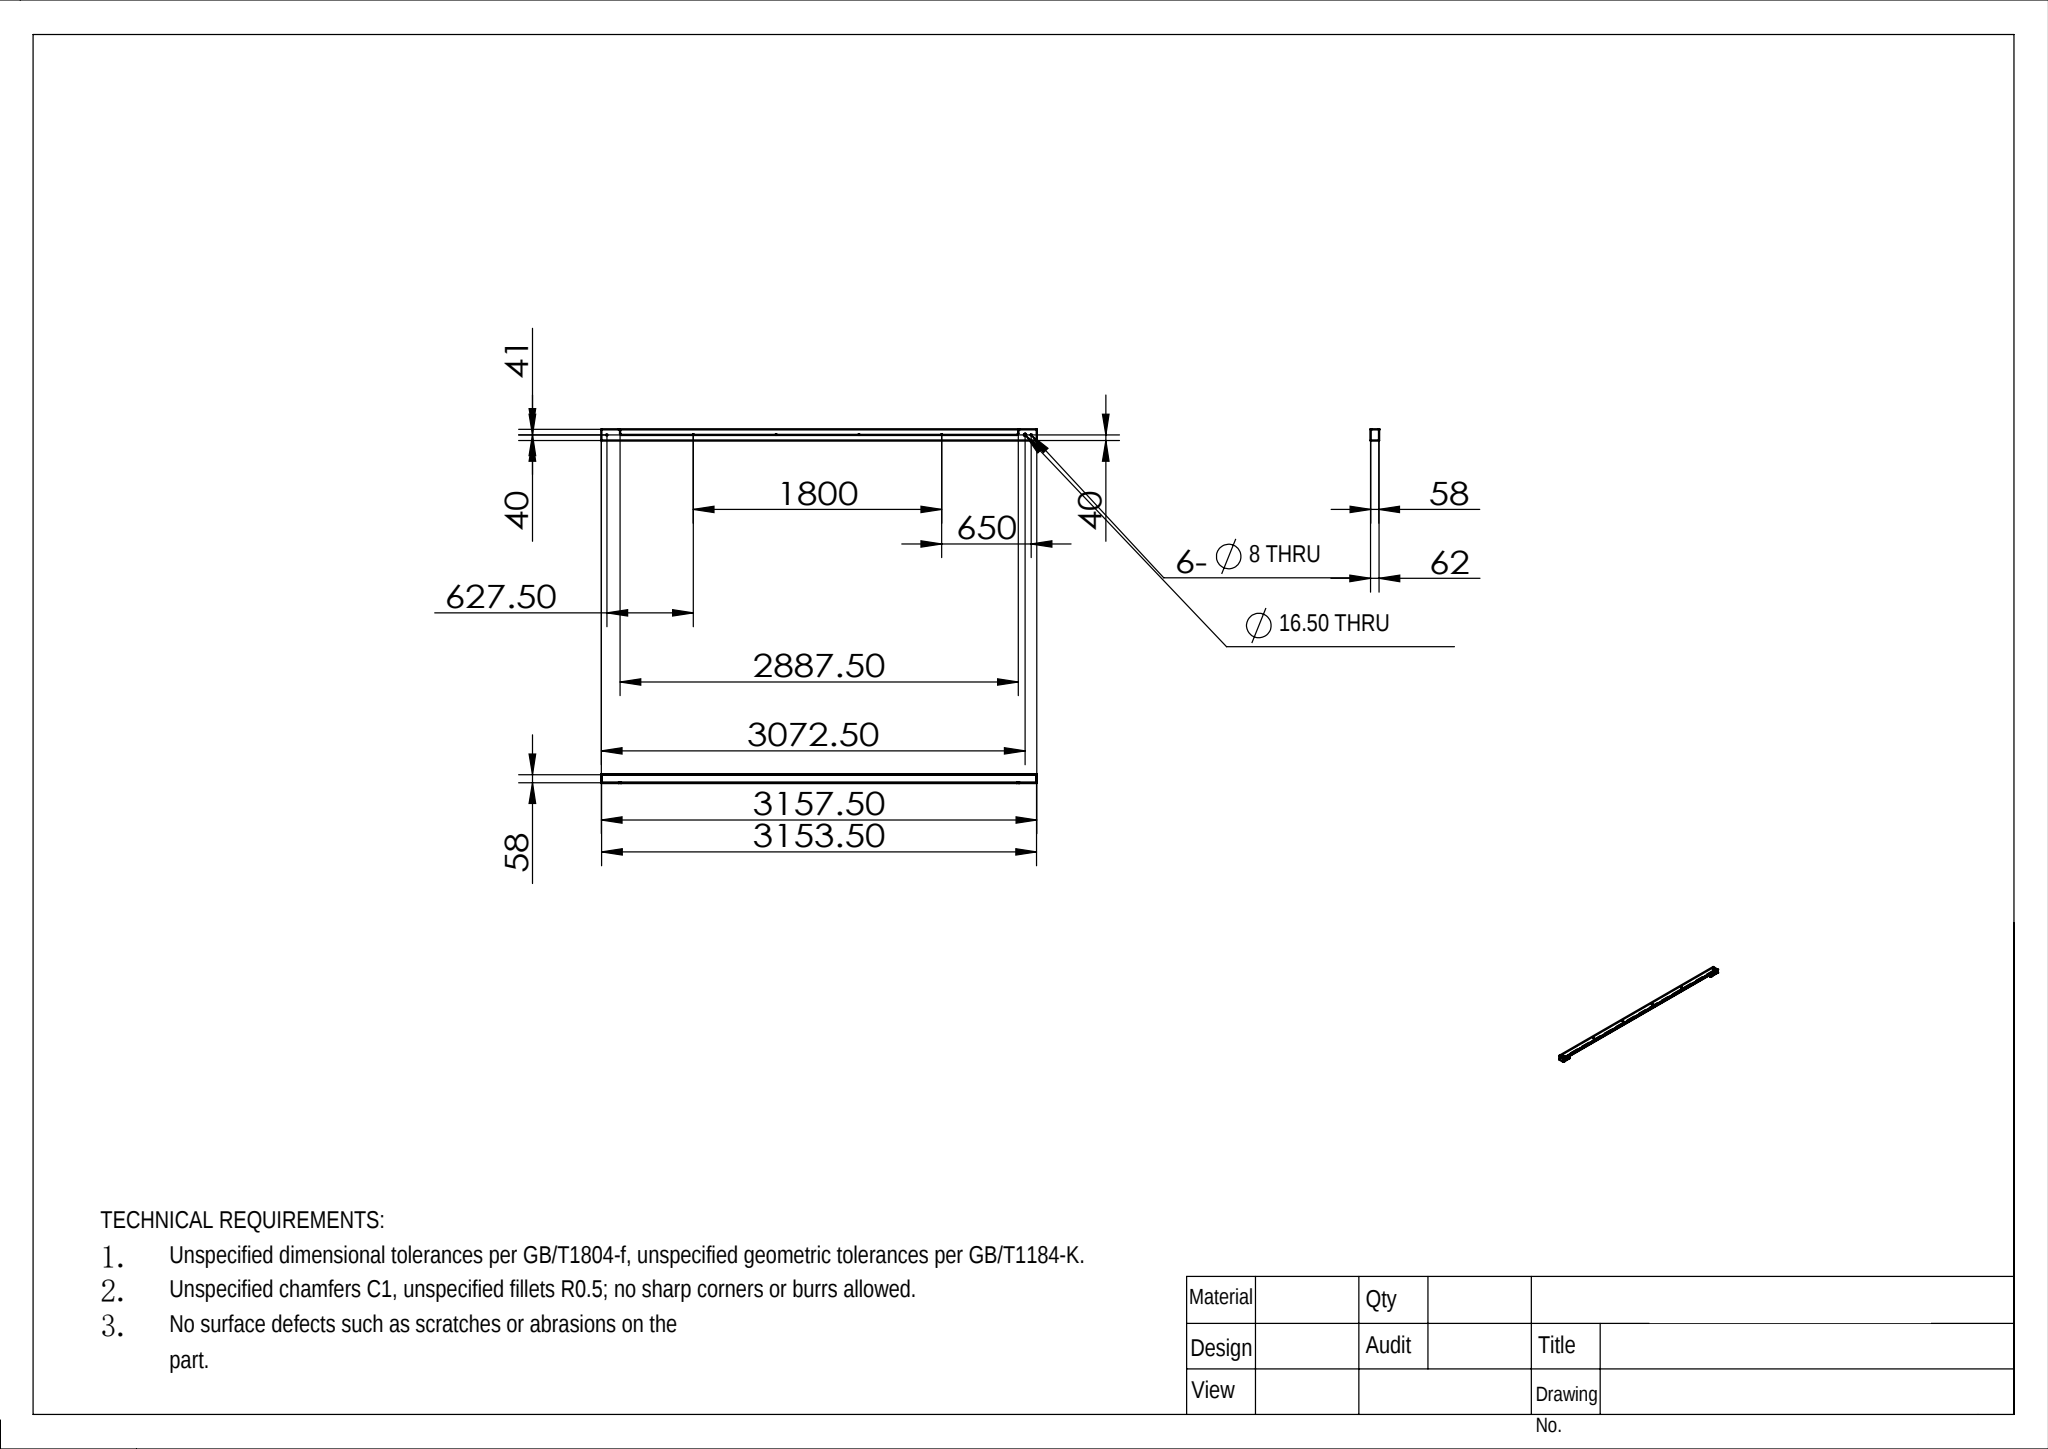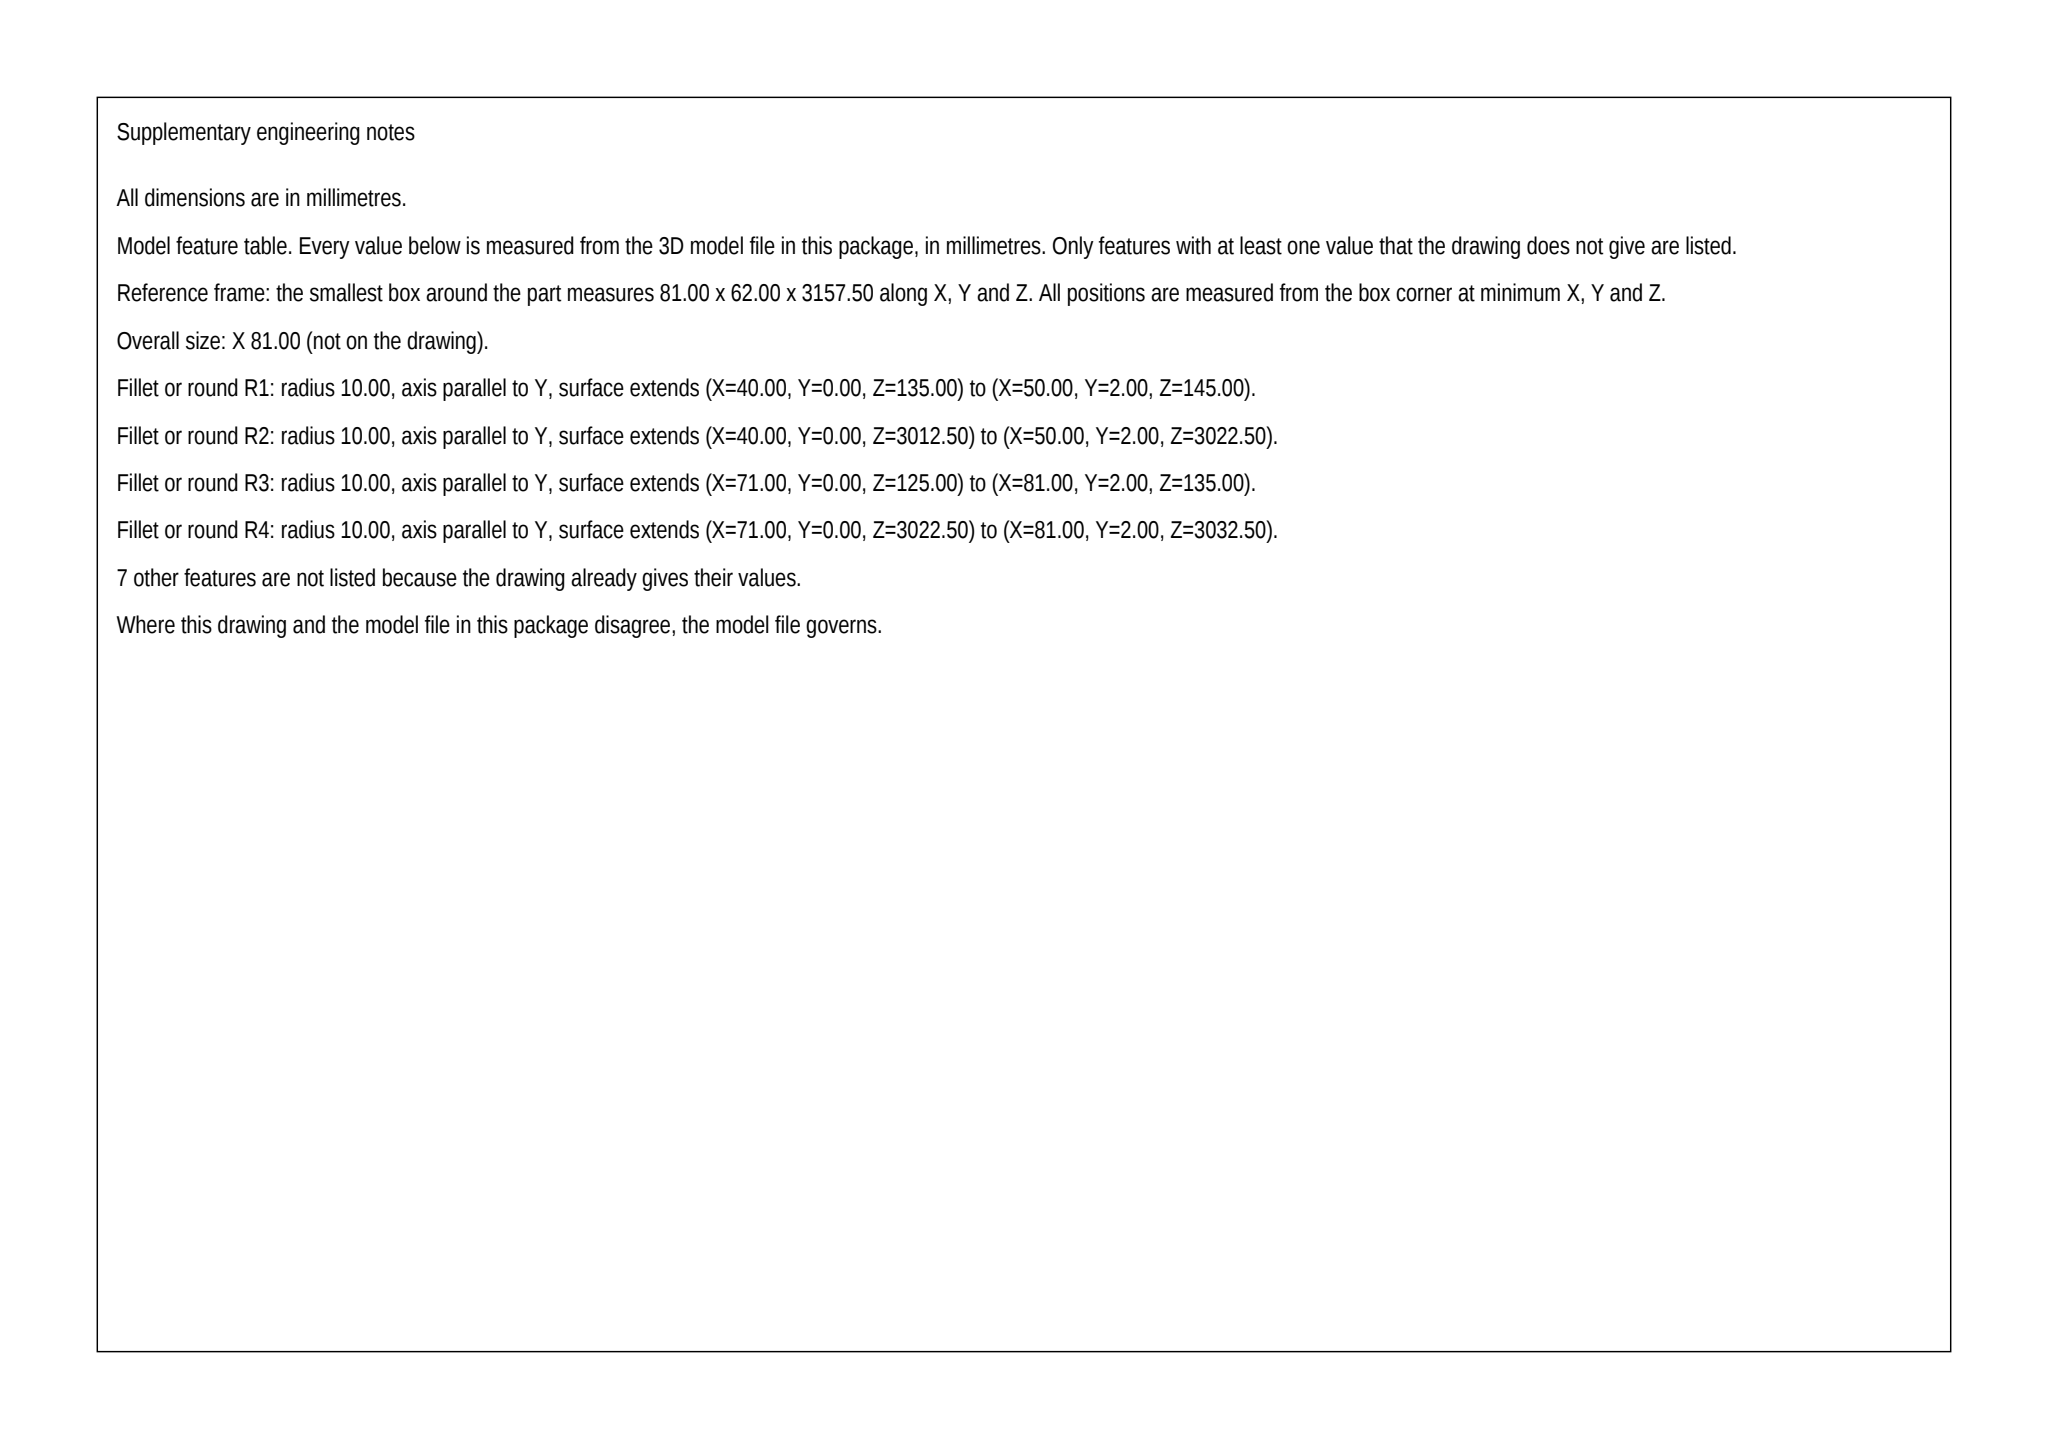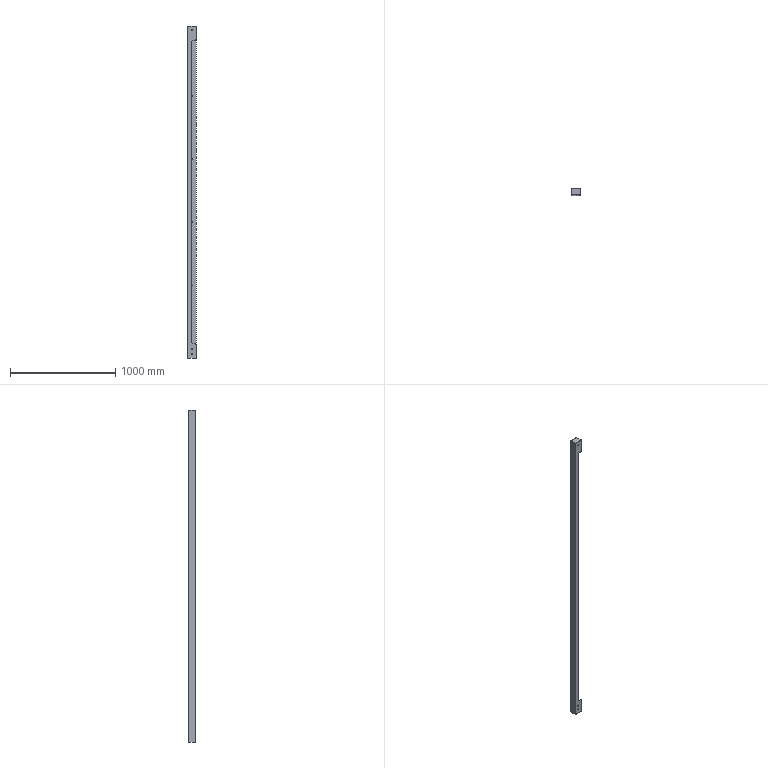Part | SolidWorks | mm | 1 solid | 40 faces | box 81 x 62 x 3157.5 mm | volume 1169389 mm3 | cylinder 22 | plane 18 | commonest cylinder face diameters 8 x16 20 x4 16.5 x2
build123d program:
from build123d import *

# Parameters (mm, degrees)
EXTRUDE_THIN1_DEPTH     = 3157.5
CUT_EXTRUDE1_DEPTH      = 10
CUT_EXTRUDE1_DEPTH_BACK = 3160.128
SKETCH4_R               = 4
SKETCH5_3_W             = 80
SKETCH5_3_H             = 62
BOSS_EXTRUDE1_DEPTH     = 2
BOSS_EXTRUDE2_START     = -3157.5
SKETCH5_3_2_W           = 80
SKETCH5_3_2_H           = 62
BOSS_EXTRUDE2_DEPTH     = 2
SKETCH6_W               = 41
SKETCH6_H               = 2887.5
CUT_EXTRUDE2_DEPTH      = 10
FILLET1_R               = 10
SKETCH7_R               = 4
CUT_EXTRUDE3_DEPTH      = 10
LPATTERN1_COUNT         = 4
LPATTERN1_PITCH         = 600
SKETCH8_R               = 8.25
CUT_EXTRUDE4_DEPTH      = 10


with BuildPart() as part:
    # Sketch1 → Extrude-Thin1 (new body)
    with BuildSketch(Plane.XY):
        Polygon((0, 1), (-81, 1), (-81, -61), (0, -61), (0, -59), (-79, -59), (-79, -1), (0, -1), align=None)
    extrude(amount=EXTRUDE_THIN1_DEPTH)

    # Sketch4 → Cut-Extrude1 (cut, two sides: drawn at the far end of the back side and taken through both)
    with BuildSketch(Plane(origin=(0, 0, 0), x_dir=(1, 0, 0), z_dir=(0, 1, 0)).offset(-CUT_EXTRUDE1_DEPTH_BACK)):
        with Locations((-41, -40)):
            Circle(SKETCH4_R)
        with Locations((-41, -3117.5)):
            Circle(SKETCH4_R)
    extrude(amount=CUT_EXTRUDE1_DEPTH + CUT_EXTRUDE1_DEPTH_BACK, mode=Mode.SUBTRACT)

    # Sketch5_3 → Boss-Extrude1 (add)
    with BuildSketch(Plane.XY.offset(3157.5)):
        with Locations((-41, -30)):
            Rectangle(SKETCH5_3_W, SKETCH5_3_H)
    extrude(amount=-BOSS_EXTRUDE1_DEPTH)

    # Sketch5_3 2 → Boss-Extrude2 (add)
    with BuildSketch(Plane.XY.offset(3157.5).offset(BOSS_EXTRUDE2_START)):
        with Locations((-41, -30)):
            Rectangle(SKETCH5_3_2_W, SKETCH5_3_2_H)
    extrude(amount=BOSS_EXTRUDE2_DEPTH)

    # Sketch6 → Cut-Extrude2 (cut)
    with BuildSketch(Plane.XZ.offset(61)):
        with Locations((-20.5, 1578.75)):
            Rectangle(SKETCH6_W, SKETCH6_H)
    extrude(amount=-CUT_EXTRUDE2_DEPTH, mode=Mode.SUBTRACT)

    # Fillet1
    fillet1_edges = [part.edges().sort_by_distance(p)[0] for p in [
        (0, -60, 3022.5),
        (0, -60, 135),
        (-41, -60, 135),
        (-41, -60, 3022.5),
    ]]
    fillet(fillet1_edges, radius=FILLET1_R)

    # Sketch7 → Cut-Extrude3 (cut)
    with BuildSketch(Plane(origin=(0, 1, 0), x_dir=(1, 0, 0), z_dir=(0, 1, 0))):
        with Locations(Location((-41, -690, 0), (0, 0, 180))):
            Circle(SKETCH7_R)
    cut_extrude3 = extrude(amount=-CUT_EXTRUDE3_DEPTH, mode=Mode.SUBTRACT)

    # LPattern1: Cut-Extrude3 ×4
    with Locations(*[(0, 0, i * LPATTERN1_PITCH) for i in range(1, LPATTERN1_COUNT)]):
        add(cut_extrude3, mode=Mode.SUBTRACT)

    # Sketch8 → Cut-Extrude4 (cut)
    with BuildSketch(Plane.XZ.offset(61)):
        with Locations((-41, 85)):
            Circle(SKETCH8_R)
    extrude(amount=-CUT_EXTRUDE4_DEPTH, mode=Mode.SUBTRACT)


solid = part.part